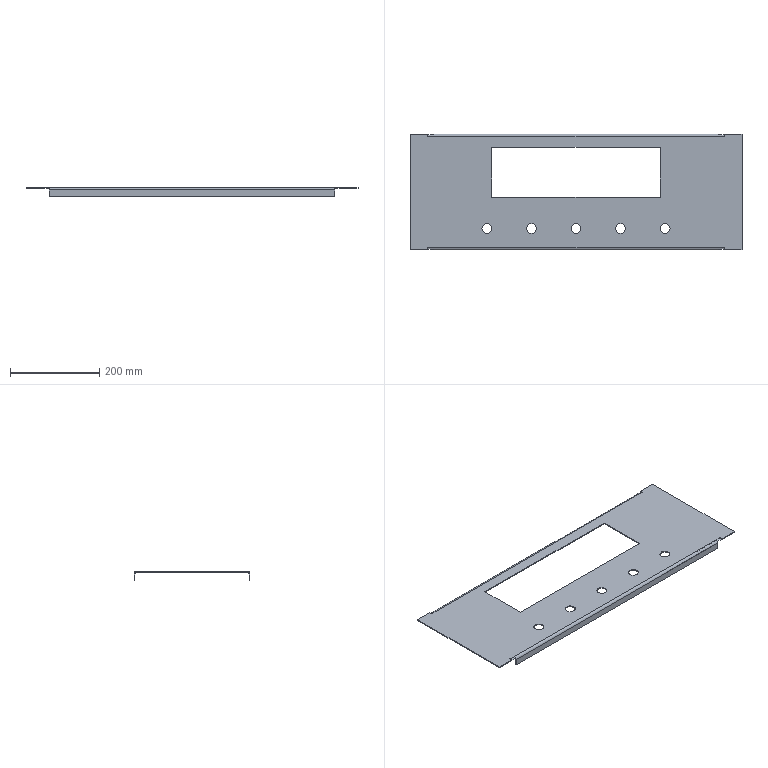Component | SolidWorks | Panel4-2 | 1 solid | 52 faces | volume 339755 mm3 | plane 38 | cylinder 14 | commonest cylinder face diameters 22 x10 11 x2 7 x2 | material Malleable Cast Iron